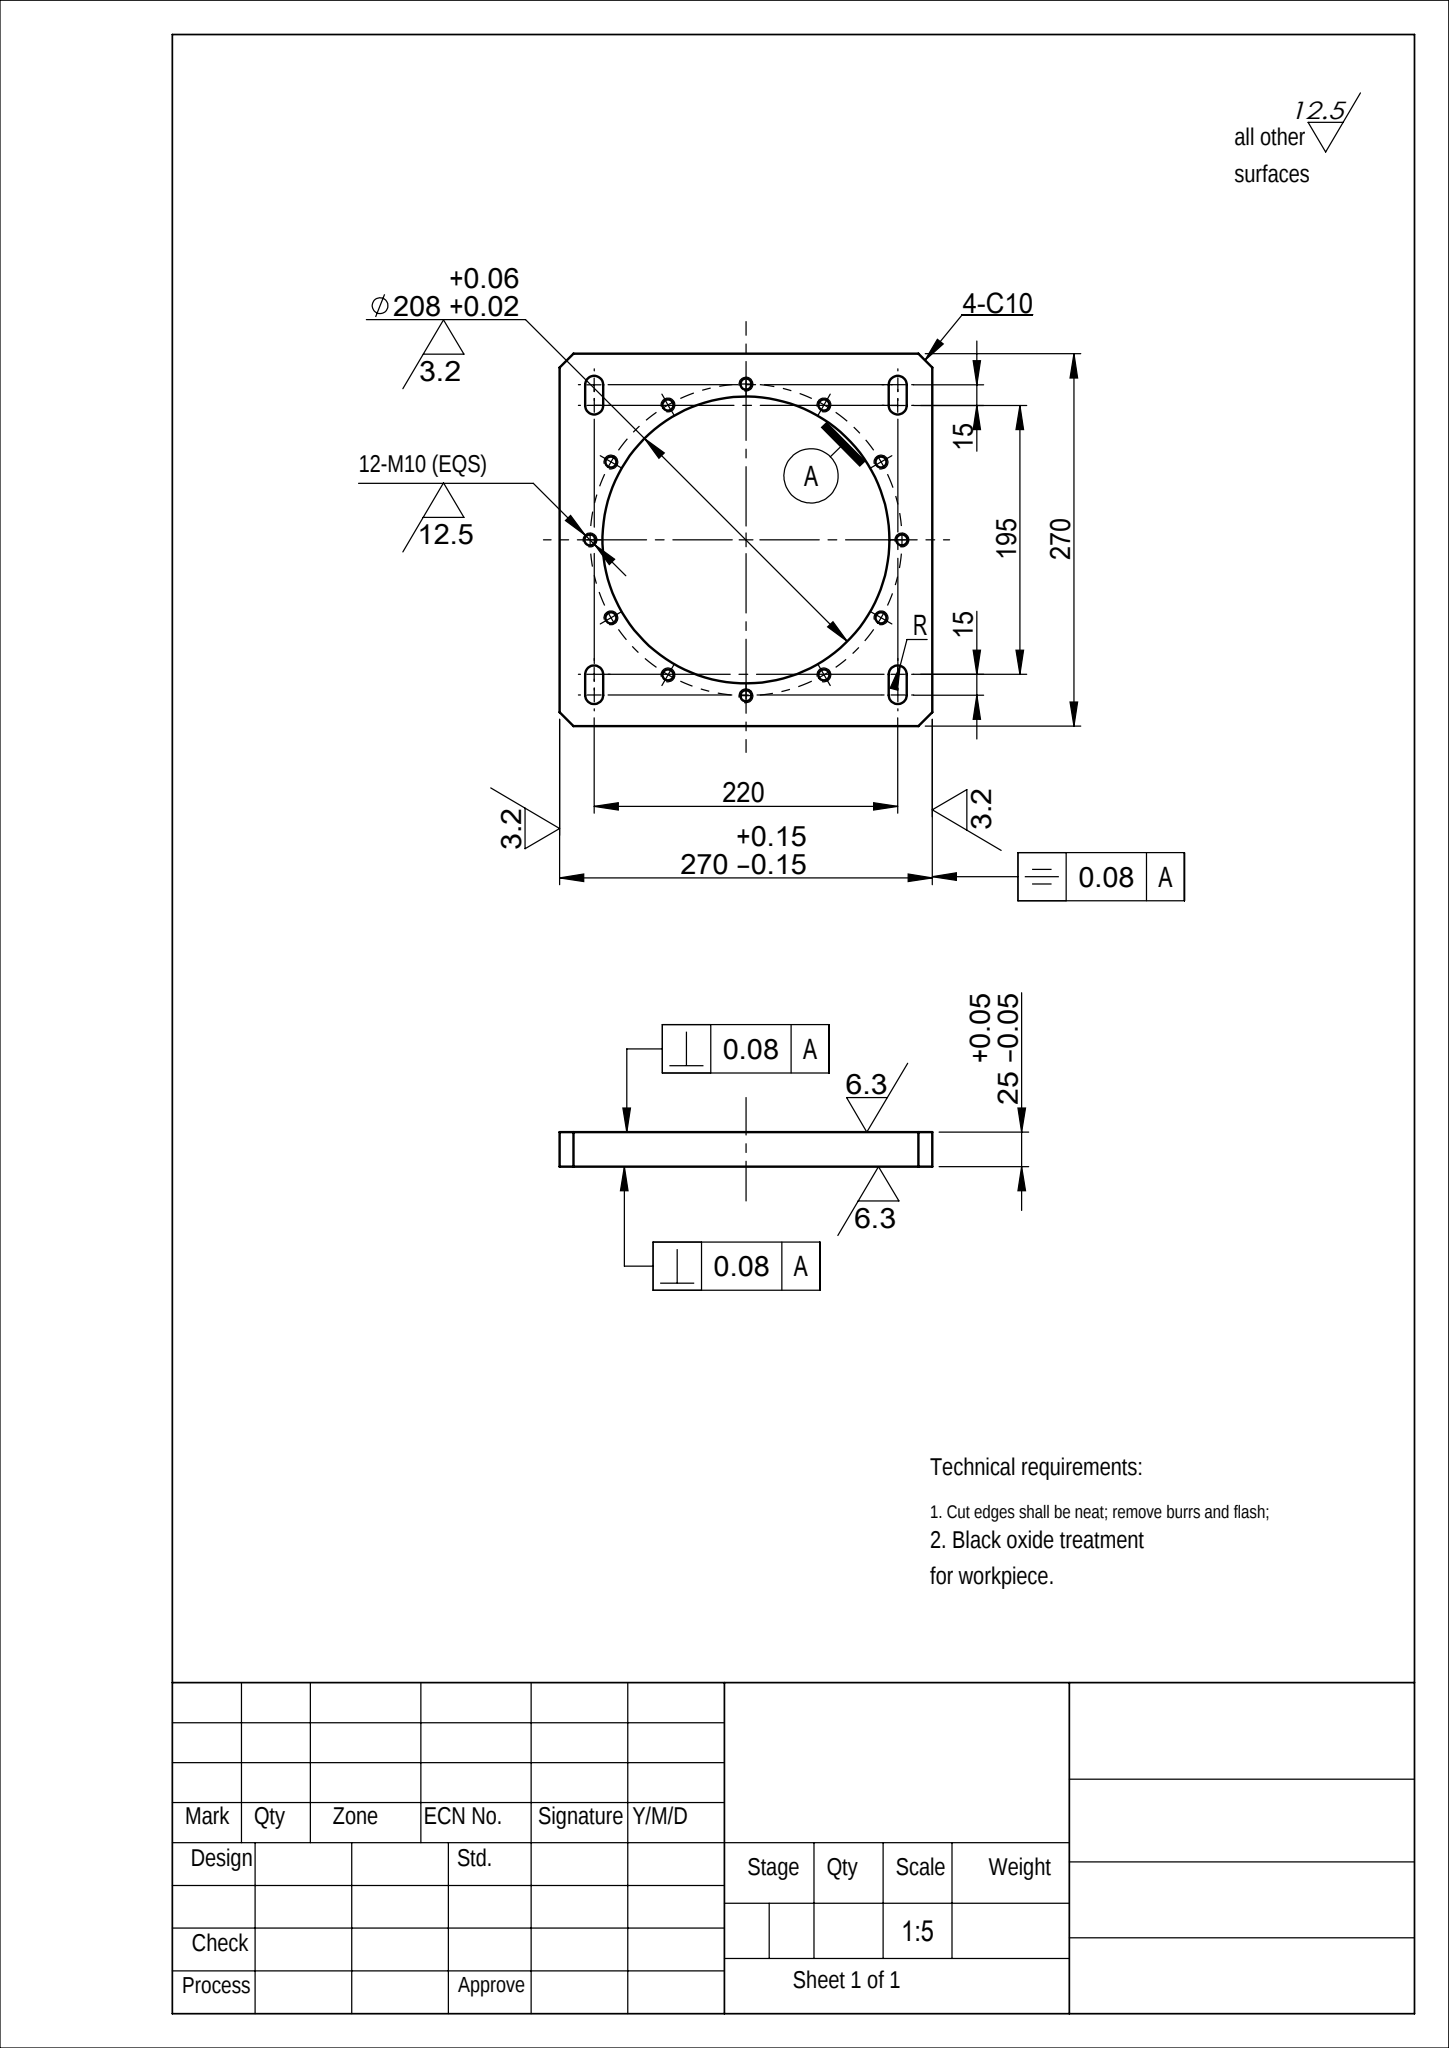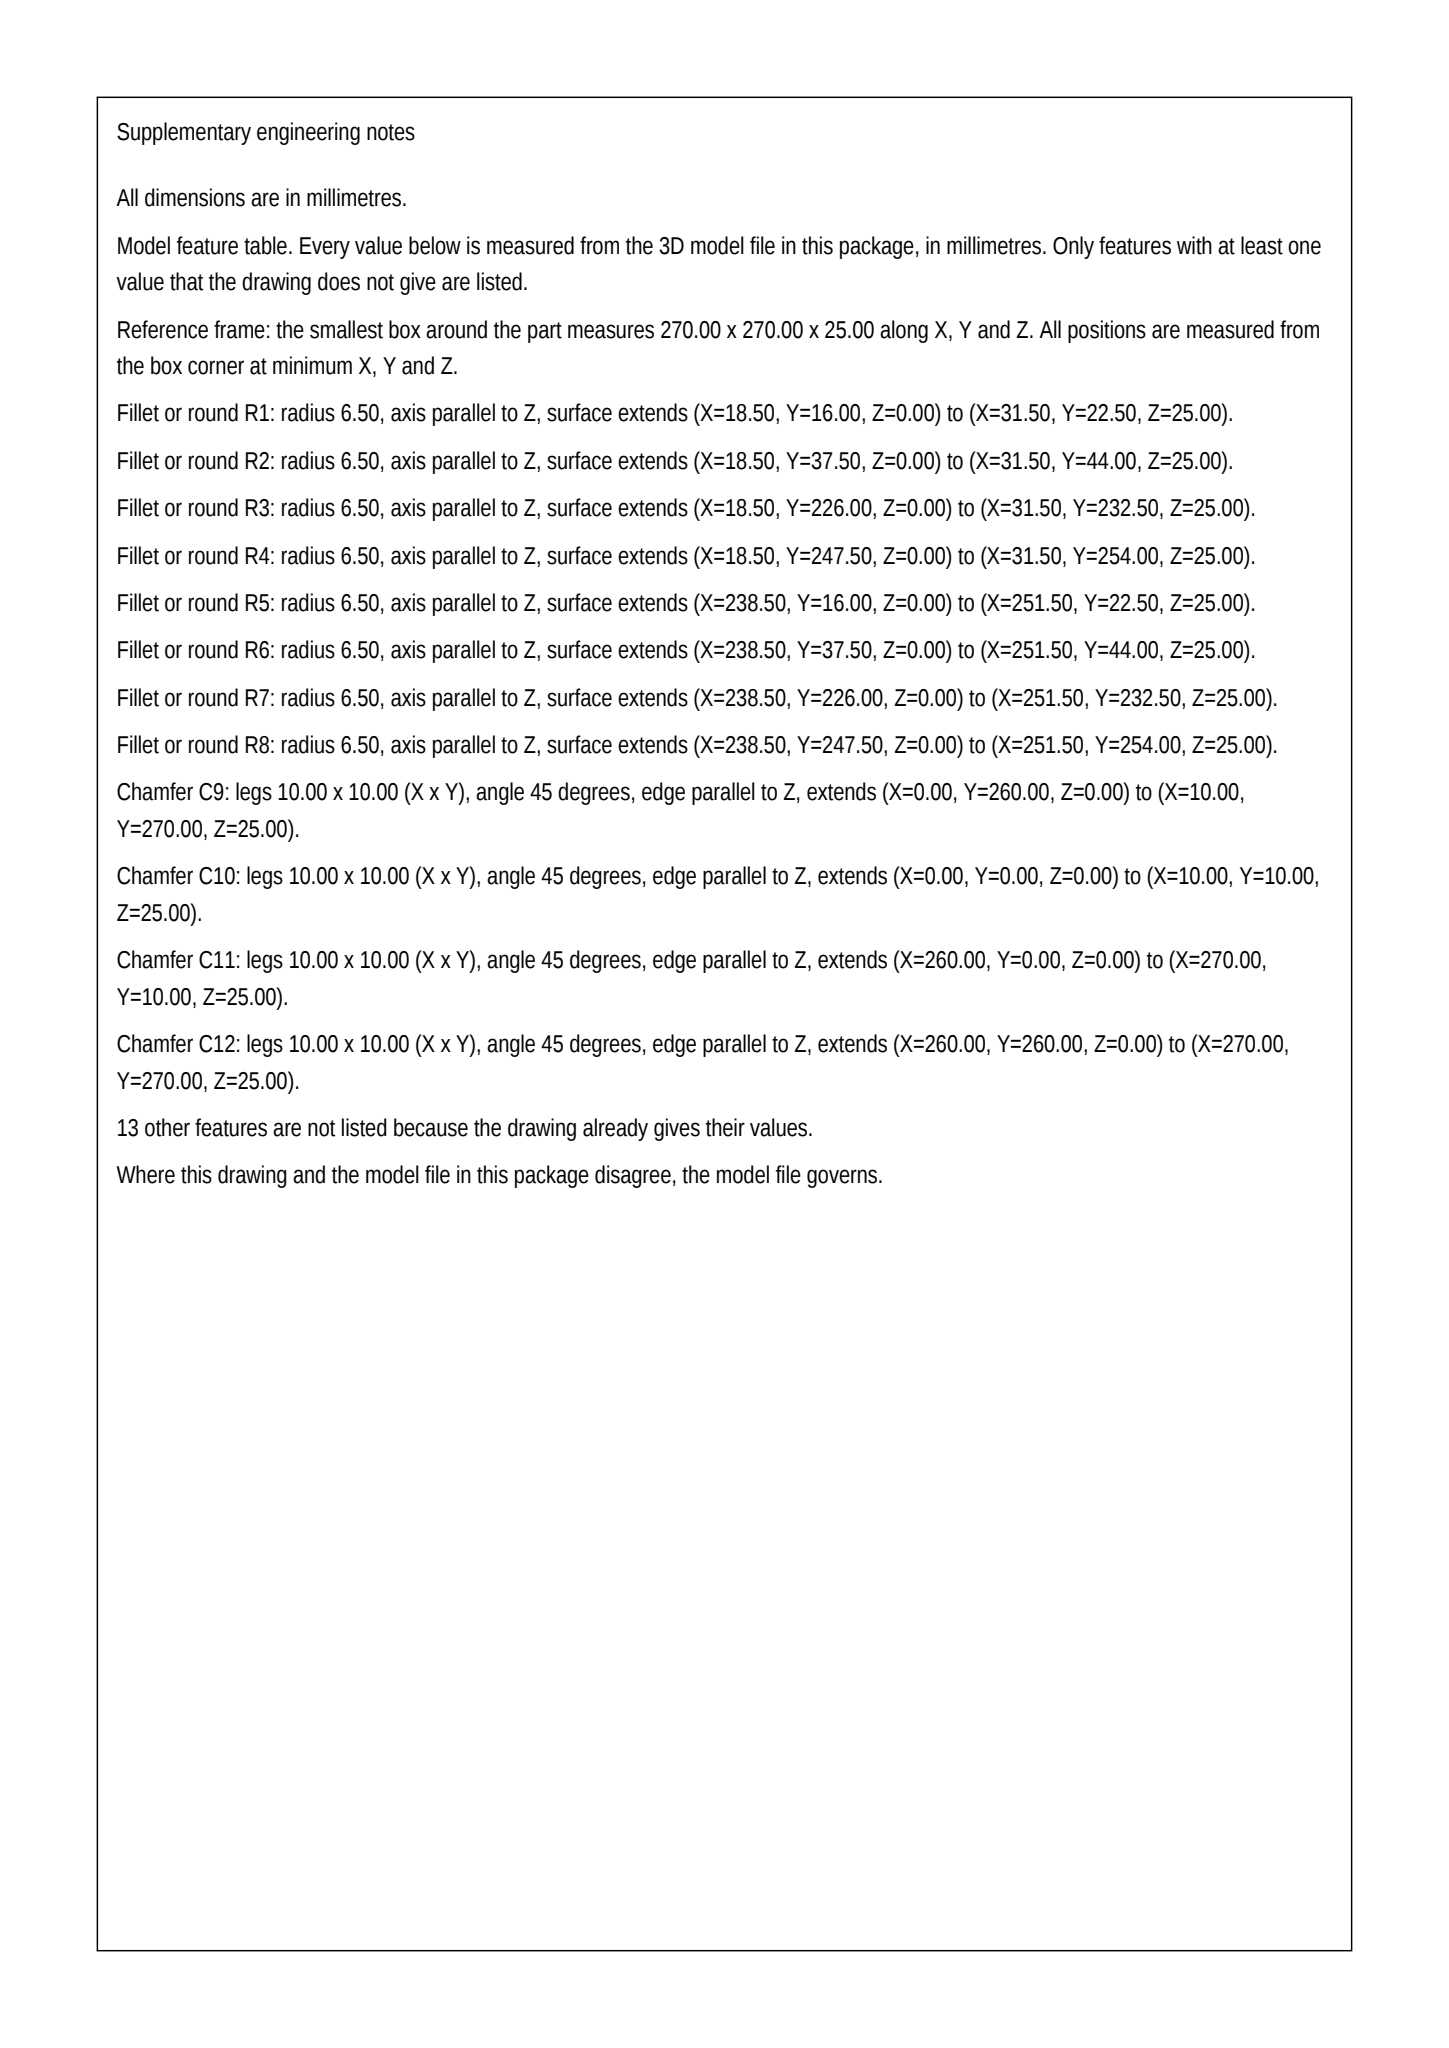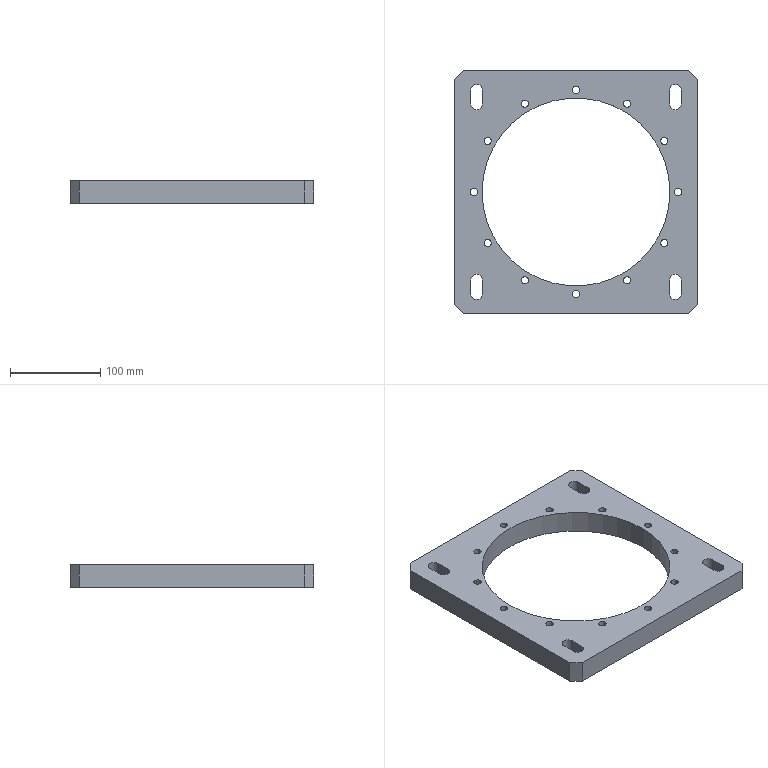Part | SolidWorks | mm | 1 solid | 52 faces | box 270 x 270 x 25 mm | volume 920160 mm3 | cylinder 34 | plane 18 | commonest cylinder face diameters 8 x24 13 x8 208 x2
build123d program:
from build123d import *

# Parameters (mm, degrees)
SKETCH1_W           = 270
SKETCH1_H           = 270
BOSS_EXTRUDE1_DEPTH = 25
SKETCH2_R           = 104
CUT_EXTRUDE1_DEPTH  = 193.549
SKETCH3_R           = 4
CUT_EXTRUDE2_DEPTH  = 193.549
CIRPATTERN1_COUNT   = 12
CHAMFER1_SIZE       = 10
CUT_EXTRUDE3_DEPTH  = 193.549


with BuildPart() as part:
    # Sketch1 → Boss-Extrude1 (new body)
    with BuildSketch(Plane.XY):
        Rectangle(SKETCH1_W, SKETCH1_H)
    extrude(amount=BOSS_EXTRUDE1_DEPTH)

    # Sketch2 → Cut-Extrude1 (cut, through all)
    with BuildSketch(Plane.XY.offset(25)):
        Circle(SKETCH2_R)
    extrude(amount=-CUT_EXTRUDE1_DEPTH, mode=Mode.SUBTRACT)

    # Sketch3 → Cut-Extrude2 (cut, through all)
    with BuildSketch(Plane.XY.offset(25)):
        with Locations((0, 113)):
            Circle(SKETCH3_R)
    cut_extrude2 = extrude(amount=-CUT_EXTRUDE2_DEPTH, mode=Mode.SUBTRACT)

    # CirPattern1: Cut-Extrude2 ×12 about axis
    cirpattern1_axis = Axis((0, 0, 0), (0, 0, 1))
    for i in range(1, CIRPATTERN1_COUNT):
        add(cut_extrude2.rotate(cirpattern1_axis, i * 360 / CIRPATTERN1_COUNT), mode=Mode.SUBTRACT)

    # Chamfer1
    chamfer1_edges = [part.edges().sort_by_distance(p)[0] for p in [
        (-135, 135, 12.5),
        (135, 135, 12.5),
        (135, -135, 12.5),
        (-135, -135, 12.5),
    ]]
    chamfer(chamfer1_edges, length=CHAMFER1_SIZE)

    # Sketch4 → Cut-Extrude3 (cut, through all)
    with BuildSketch(Plane.XY.offset(25)):
        with BuildLine():
            Line((-116.5, 97.5), (-116.5, 112.5))
            ThreePointArc((-116.5, 112.5), (-110, 119), (-103.5, 112.5))
            Line((-103.5, 112.5), (-103.5, 97.5))
            ThreePointArc((-103.5, 97.5), (-110, 91), (-116.5, 97.5))
        make_face()
        with BuildLine():
            Line((116.5, 97.5), (116.5, 112.5))
            ThreePointArc((116.5, 112.5), (110, 119), (103.5, 112.5))
            Line((103.5, 112.5), (103.5, 97.5))
            ThreePointArc((103.5, 97.5), (110, 91), (116.5, 97.5))
        make_face()
        with BuildLine():
            Line((-116.5, -112.5), (-116.5, -97.5))
            ThreePointArc((-116.5, -97.5), (-110, -91), (-103.5, -97.5))
            Line((-103.5, -97.5), (-103.5, -112.5))
            ThreePointArc((-103.5, -112.5), (-110, -119), (-116.5, -112.5))
        make_face()
        with BuildLine():
            Line((116.5, -112.5), (116.5, -97.5))
            ThreePointArc((116.5, -97.5), (110, -91), (103.5, -97.5))
            Line((103.5, -97.5), (103.5, -112.5))
            ThreePointArc((103.5, -112.5), (110, -119), (116.5, -112.5))
        make_face()
    extrude(amount=-CUT_EXTRUDE3_DEPTH, mode=Mode.SUBTRACT)


solid = part.part